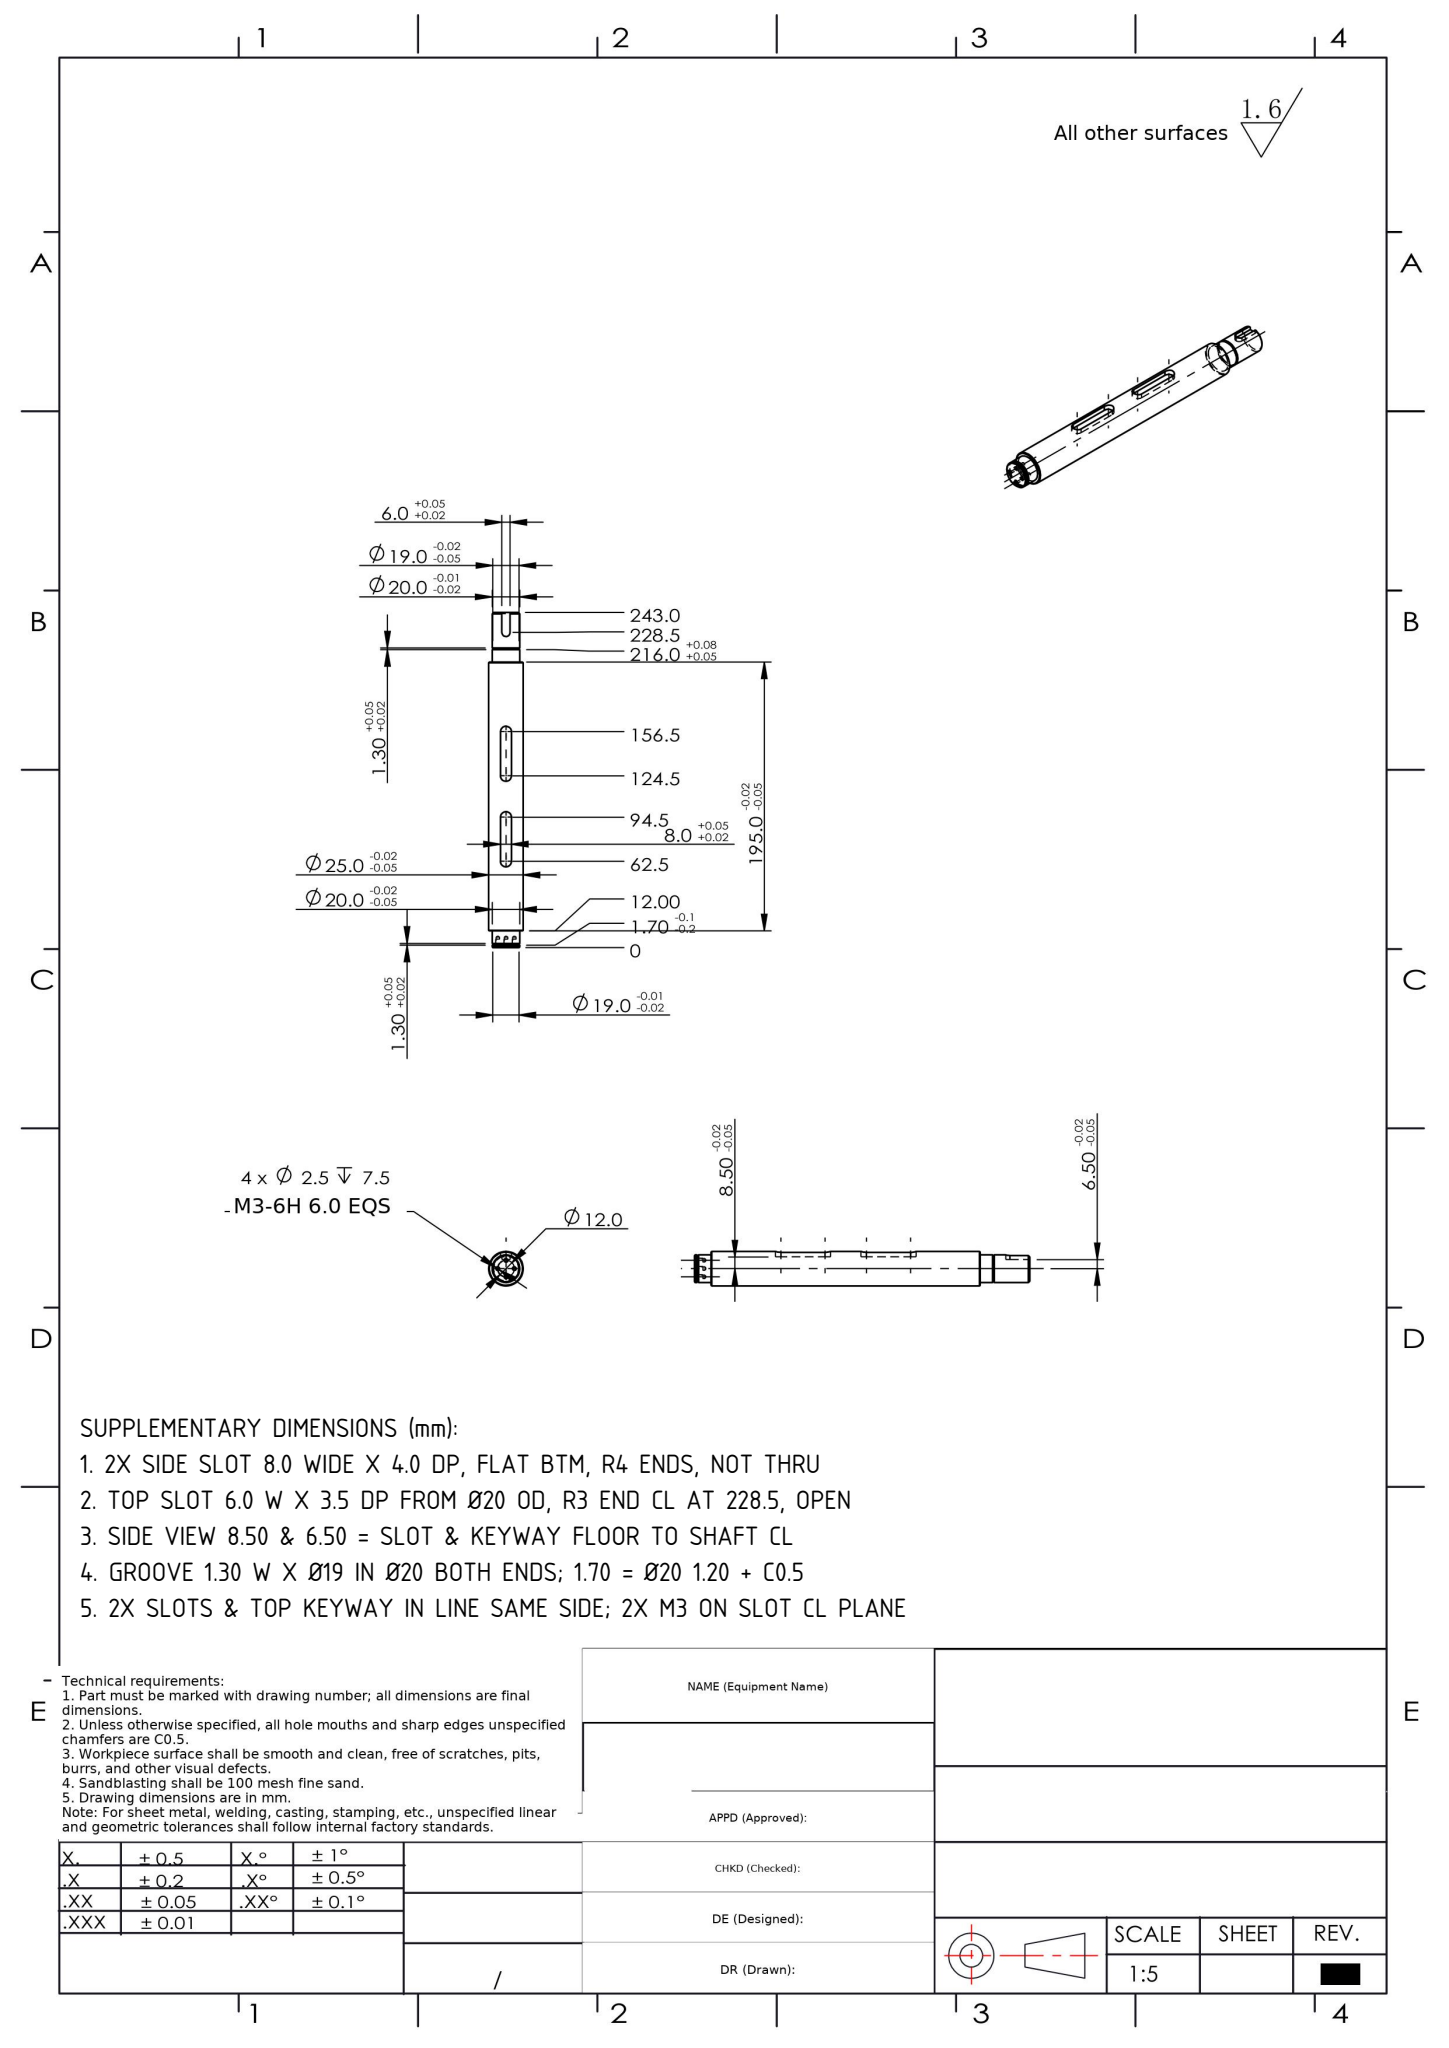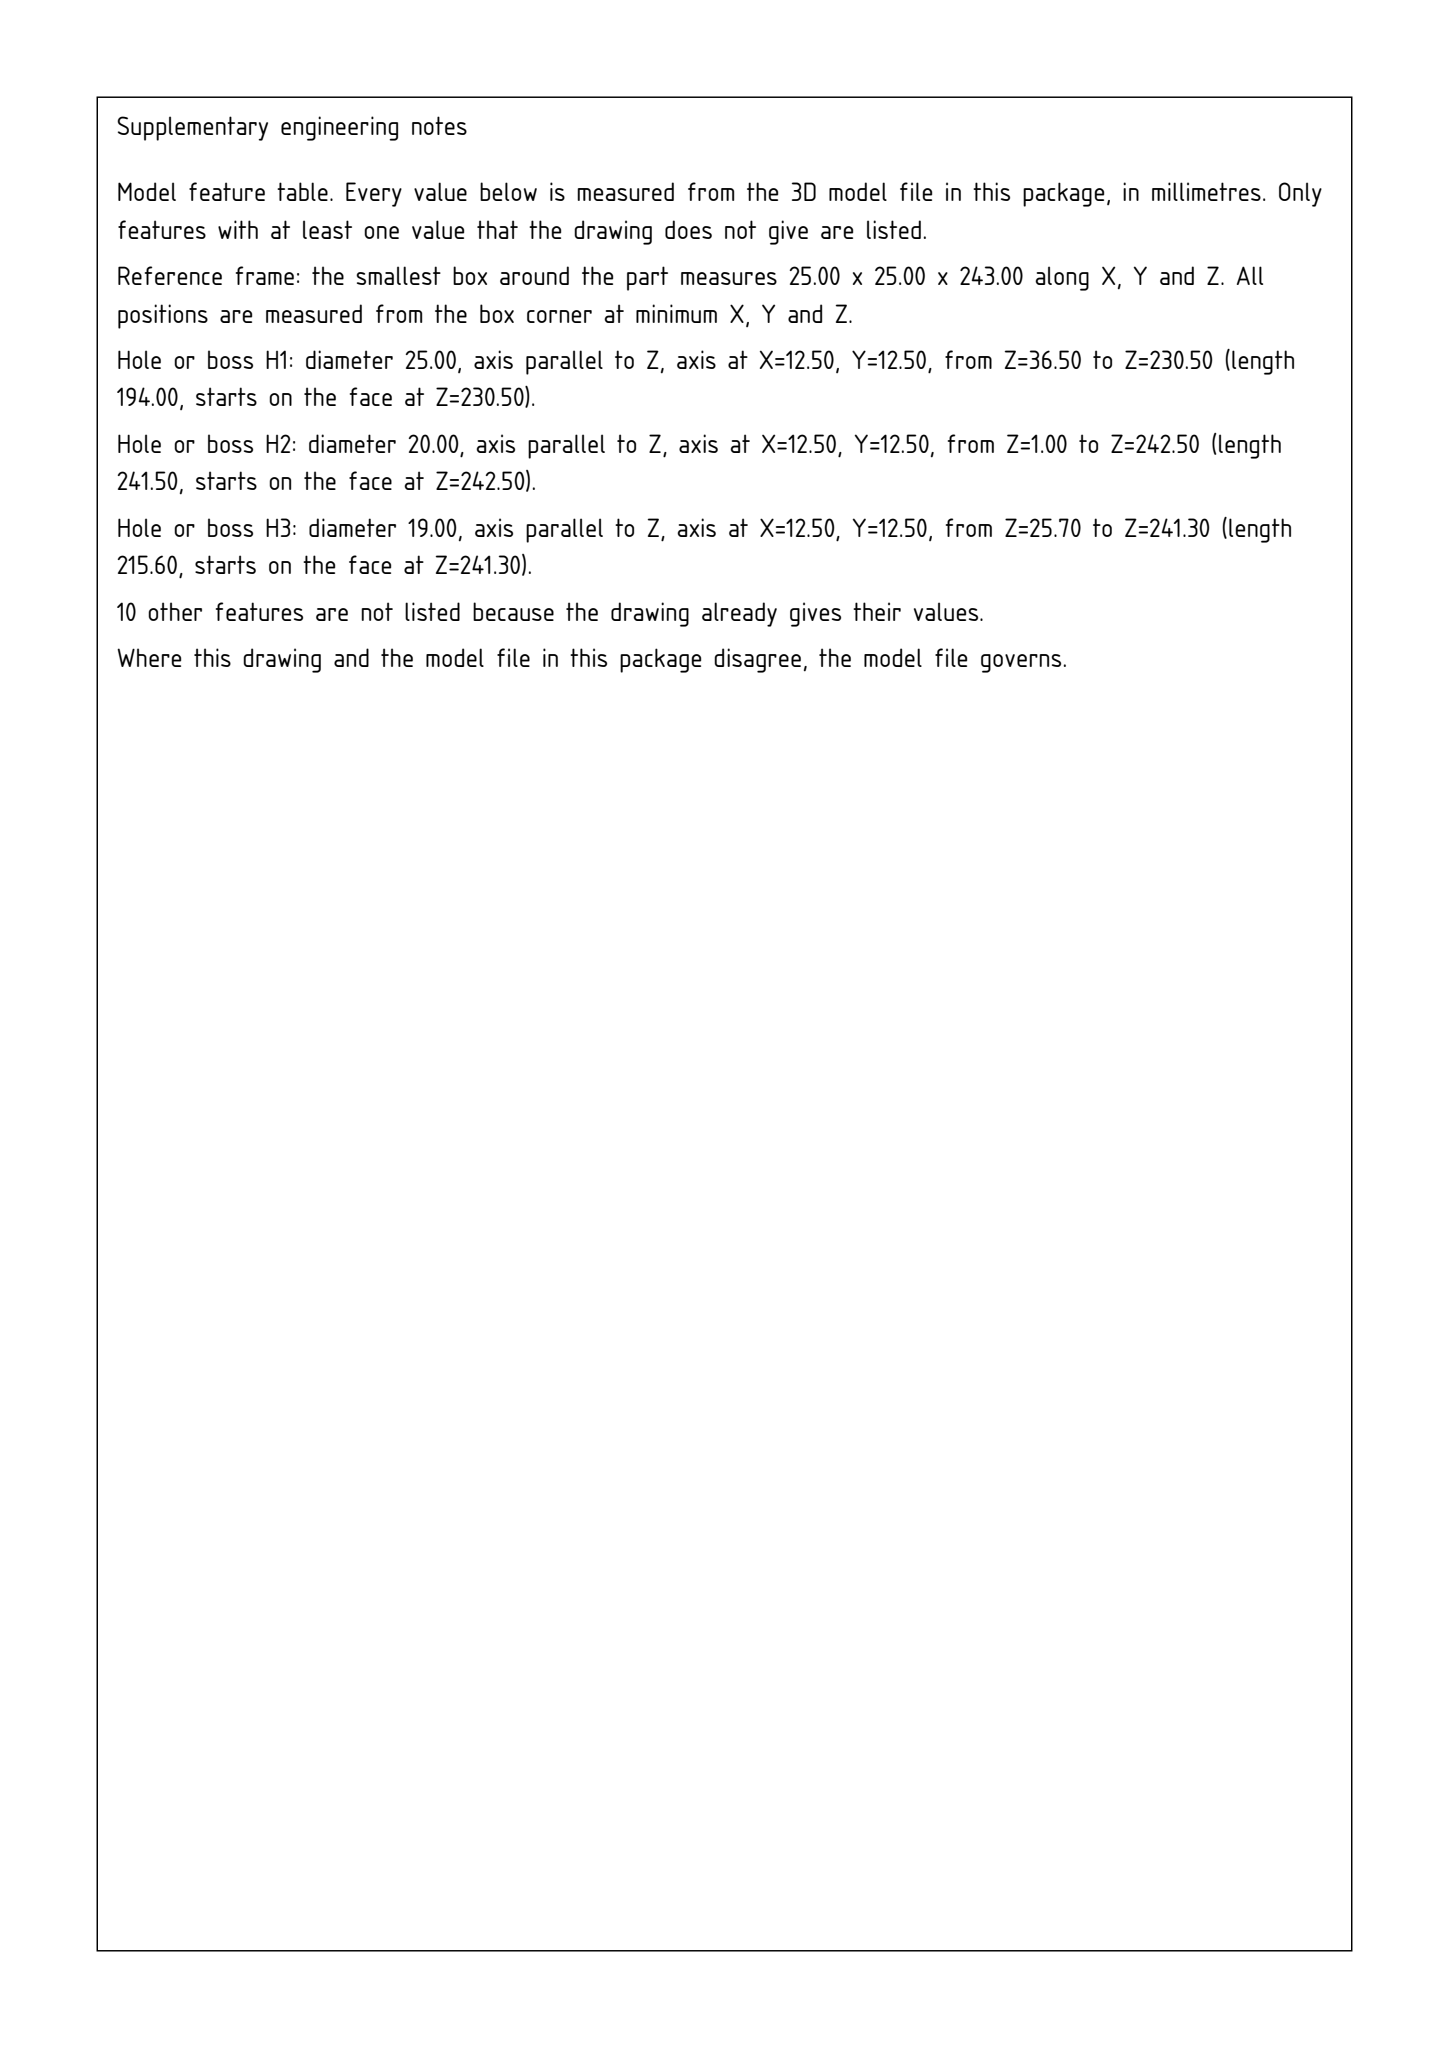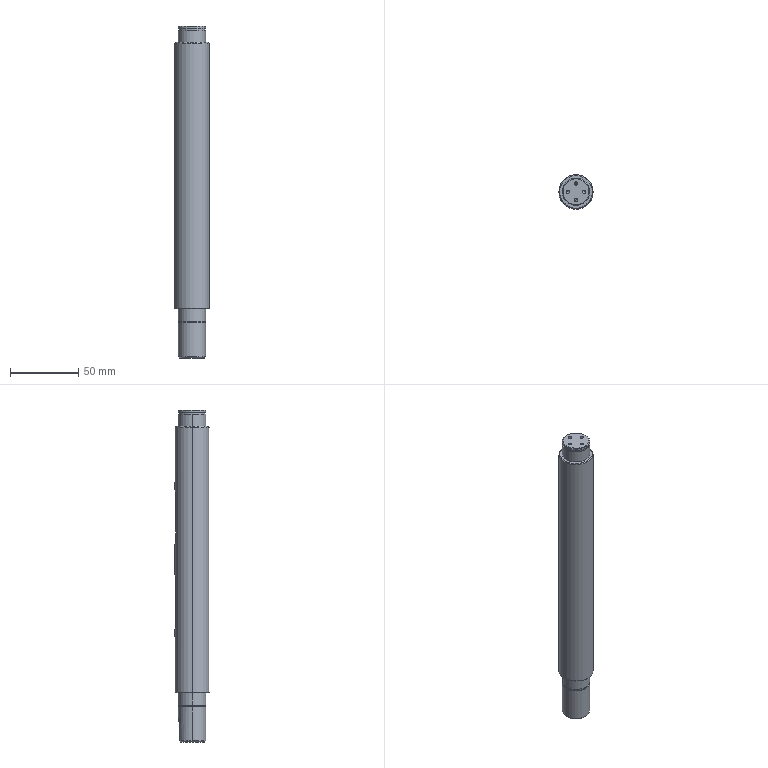Part | SolidWorks | mm | 1 solid | 64 faces | box 25 x 25 x 243 mm | volume 107852 mm3 | cylinder 30 | cone 17 | plane 17 | commonest cylinder face diameters 2.5 x8 20 x8 8 x6 19 x4 25 x2 6 x2